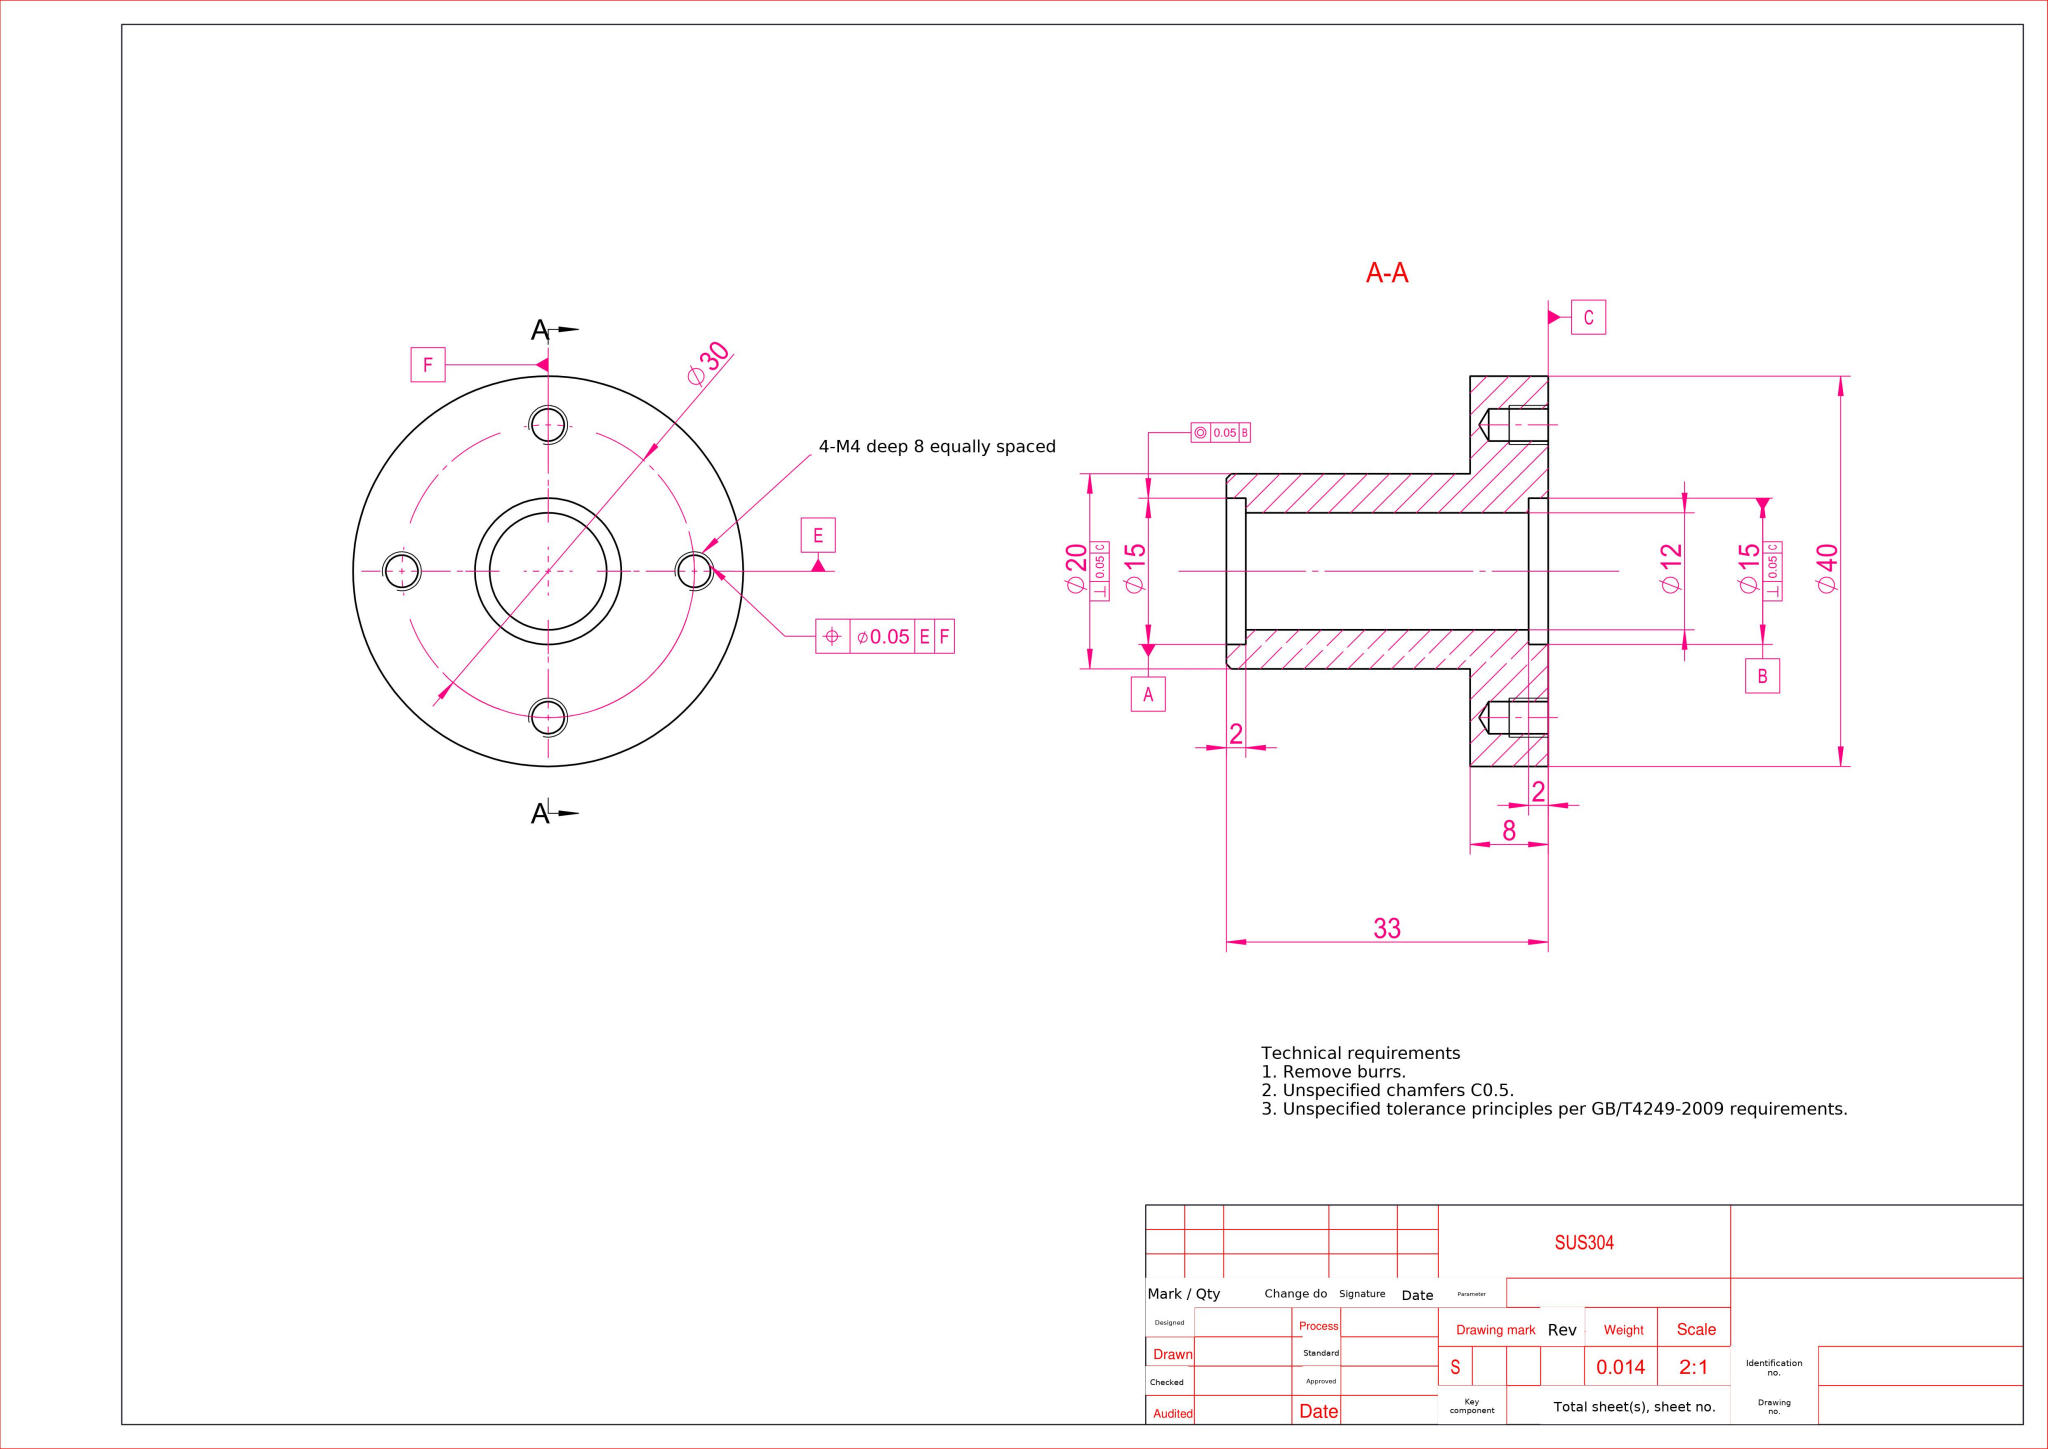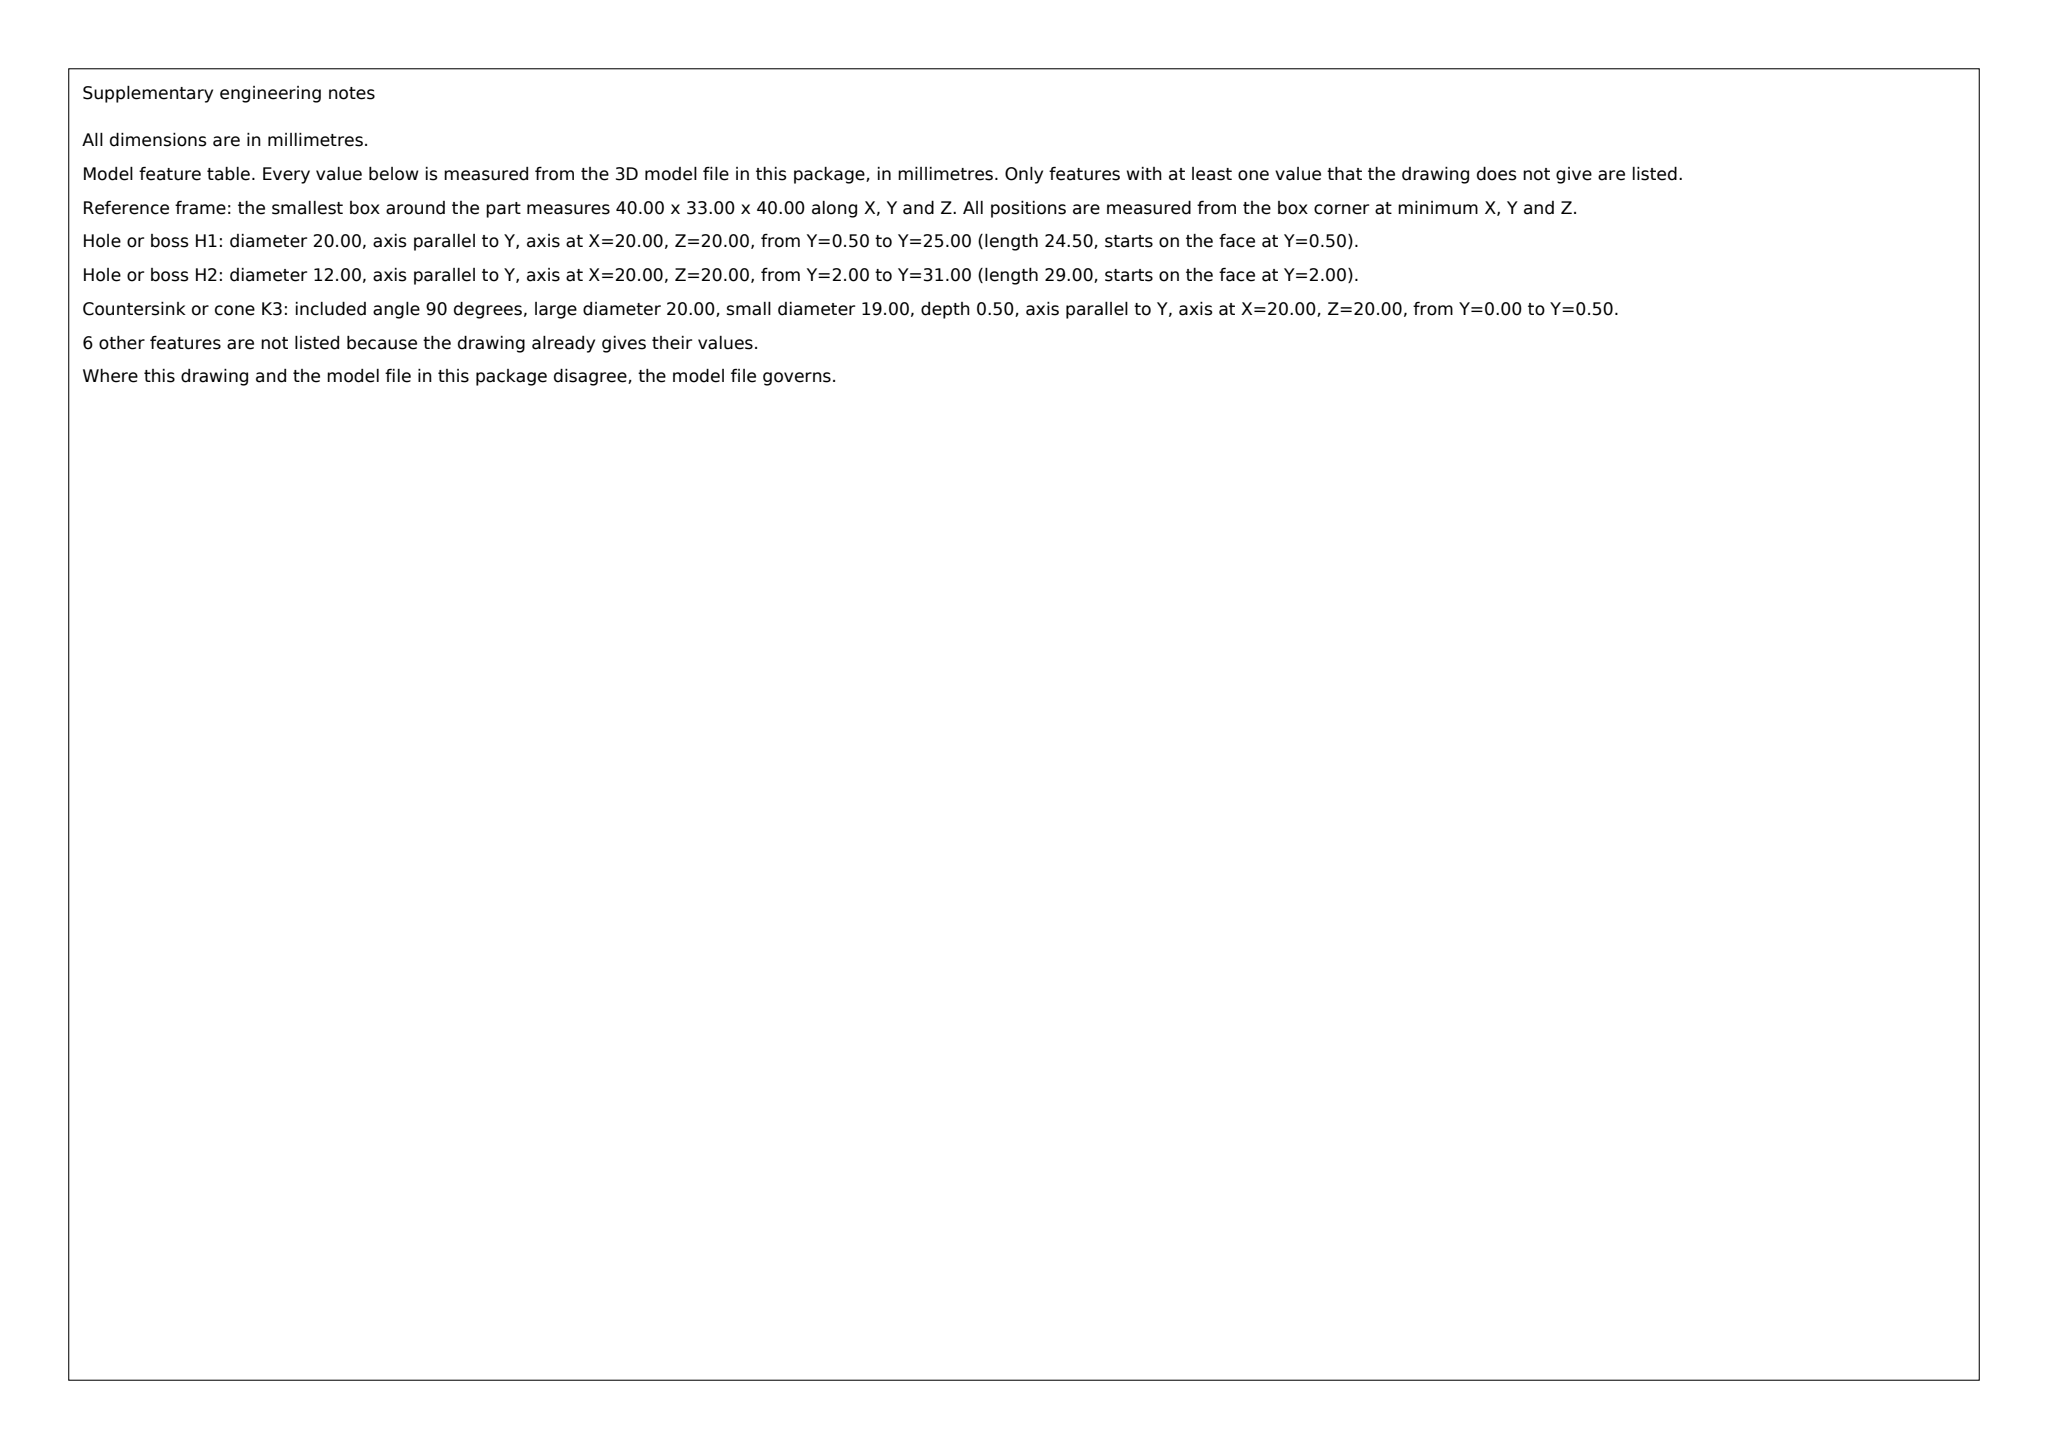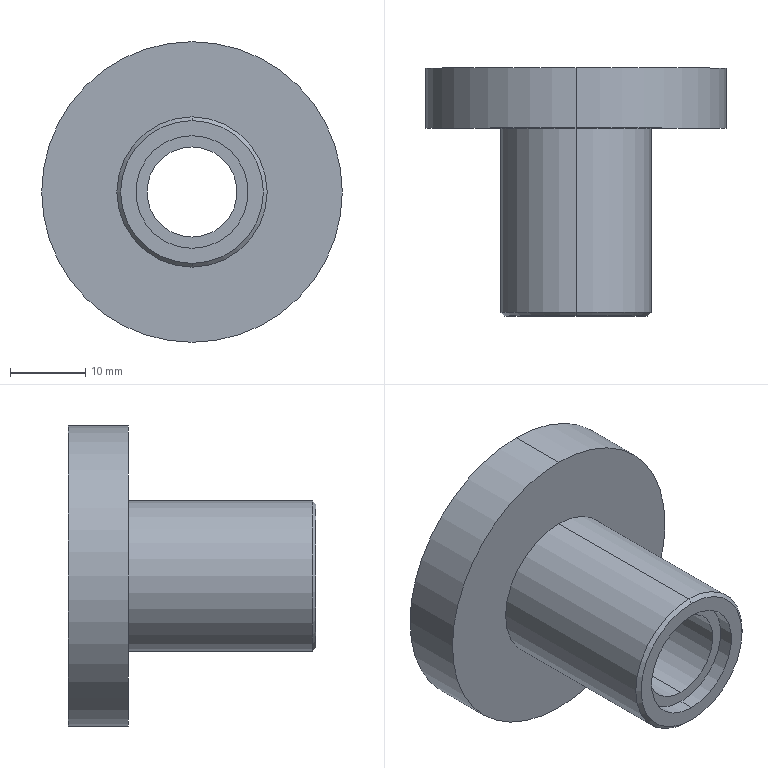Part | SolidWorks | mm | material SUS304 | 1 solid | 33 faces | box 40 x 33 x 40 mm | volume 13693 mm3 | cylinder 18 | cone 10 | plane 5 | commonest cylinder face diameters 3.3 x8 15 x4 40 x2 20 x2 12 x2
build123d program:
from build123d import *

# Parameters (mm, degrees)
SKETCH2_R             = 6
CUT_EXTRUDE1_DEPTH    = 44.463
SKETCH3_R             = 7.5
CUT_EXTRUDE2_DEPTH    = 2
CHAMFER1_SIZE         = 0.5
CUT_EXTRUDE3_START    = -2
SKETCH4_R             = 7.5
CUT_EXTRUDE3_DEPTH    = 2
M4_TAPPED_HOLE3_D     = 3.3
M4_TAPPED_HOLE3_DEPTH = 6.1
M4_TAPPED_HOLE3_TIP   = 0.9914


with BuildPart() as part:
    # Sketch1 → Revolve1 (revolve)
    with BuildSketch(Plane.XY, mode=Mode.PRIVATE) as revolve1_sk:
        Polygon((0, 0), (10, 0), (10, 25), (20, 25), (20, 33), (0, 33), align=None)
    revolve(revolve1_sk.sketch.rotate(Axis((0, 65.527, 0), (0, -1, 0)), 90), axis=Axis((0, 65.527, 0), (0, -1, 0)))

    # Sketch2 → Cut-Extrude1 (cut, through all)
    with BuildSketch(Plane.XZ):
        with Locations(Location((0, 0, 0), (0, 0, 270))):
            Circle(SKETCH2_R)
    extrude(amount=-CUT_EXTRUDE1_DEPTH, mode=Mode.SUBTRACT)

    # Sketch3 → Cut-Extrude2 (cut)
    with BuildSketch(Plane.XZ):
        with Locations(Location((0, 0, 0), (0, 0, 270))):
            Circle(SKETCH3_R)
    extrude(amount=-CUT_EXTRUDE2_DEPTH, mode=Mode.SUBTRACT)

    # Chamfer1
    chamfer1_edges = [part.edges().sort_by_distance(p)[0] for p in [
        (0, 0, -10),
    ]]
    chamfer(chamfer1_edges, length=CHAMFER1_SIZE)

    # Sketch4 → Cut-Extrude3 (cut)
    with BuildSketch(Plane(origin=(0, 33, 0), x_dir=(1, 0, 0), z_dir=(0, 1, 0)).offset(CUT_EXTRUDE3_START)):
        with Locations(Location((0, 0, 0), (0, 0, 90))):
            Circle(SKETCH4_R)
    extrude(amount=CUT_EXTRUDE3_DEPTH, mode=Mode.SUBTRACT)

    # M4 Tapped Hole3
    with Locations(Plane(origin=(0, 33, 0), x_dir=(1, 0, 0), z_dir=(0, 1, 0))):
        with Locations((0, 15), (15, 0), (0, -15), (-15, 0), (0, 0)):
            Hole(M4_TAPPED_HOLE3_D / 2, depth=M4_TAPPED_HOLE3_DEPTH)
            with Locations((0, 0, -(M4_TAPPED_HOLE3_DEPTH + M4_TAPPED_HOLE3_TIP / 2))):  # 118° drill point
                Cone(0, M4_TAPPED_HOLE3_D / 2, M4_TAPPED_HOLE3_TIP, mode=Mode.SUBTRACT)


solid = part.part
STEP:
#1=CARTESIAN_POINT('',(0.,26.9,-16.65));
#2=VERTEX_POINT('',#1);
#3=CARTESIAN_POINT('',(0.,26.9,-13.35));
#4=VERTEX_POINT('',#3);
#5=CARTESIAN_POINT('',(0.,26.9,-15.));
#6=DIRECTION('',(-0.,1.,0.));
#7=DIRECTION('',(0.,0.,1.));
#8=AXIS2_PLACEMENT_3D('',#5,#6,#7);
#9=CIRCLE('',#8,1.65);
#10=EDGE_CURVE('',#2,#4,#9,.T.);
#11=ORIENTED_EDGE('',*,*,#10,.F.);
#12=CARTESIAN_POINT('',(0.,33.,-16.65));
#13=VERTEX_POINT('',#12);
#14=CARTESIAN_POINT('',(0.,33.,-16.65));
#15=DIRECTION('',(-0.,1.,0.));
#16=VECTOR('',#15,1000.);
#17=LINE('',#14,#16);
#18=EDGE_CURVE('',#2,#13,#17,.T.);
#19=ORIENTED_EDGE('',*,*,#18,.T.);
#20=CARTESIAN_POINT('',(0.,33.,-13.35));
#21=VERTEX_POINT('',#20);
#22=CARTESIAN_POINT('',(0.,33.,-15.));
#23=DIRECTION('',(-0.,1.,0.));
#24=DIRECTION('',(0.,0.,1.));
#25=AXIS2_PLACEMENT_3D('',#22,#23,#24);
#26=CIRCLE('',#25,1.65);
#27=EDGE_CURVE('',#13,#21,#26,.T.);
#28=ORIENTED_EDGE('',*,*,#27,.T.);
#29=CARTESIAN_POINT('',(0.,33.,-13.35));
#30=DIRECTION('',(-0.,1.,0.));
#31=VECTOR('',#30,1000.);
#32=LINE('',#29,#31);
#33=EDGE_CURVE('',#4,#21,#32,.T.);
#34=ORIENTED_EDGE('',*,*,#33,.F.);
#35=EDGE_LOOP('',(#11,#19,#28,#34));
#36=FACE_OUTER_BOUND('',#35,.T.);
#37=CARTESIAN_POINT('',(0.,33.,-15.));
#38=DIRECTION('',(-0.,1.,0.));
#39=DIRECTION('',(0.,0.,1.));
#40=AXIS2_PLACEMENT_3D('',#37,#38,#39);
#41=CYLINDRICAL_SURFACE('',#40,1.65);
#42=ADVANCED_FACE('',(#36),#41,.F.);
#43=CARTESIAN_POINT('',(-0.,25.909,-15.));
#44=VERTEX_POINT('',#43);
#45=CARTESIAN_POINT('',(0.,26.9,-13.35));
#46=DIRECTION('',(-0.,0.515,0.8572));
#47=VECTOR('',#46,1000.);
#48=LINE('',#45,#47);
#49=EDGE_CURVE('',#44,#4,#48,.T.);
#50=ORIENTED_EDGE('',*,*,#49,.F.);
#51=CARTESIAN_POINT('',(0.,26.9,-16.65));
#52=DIRECTION('',(0.,0.515,-0.8572));
#53=VECTOR('',#52,1000.);
#54=LINE('',#51,#53);
#55=EDGE_CURVE('',#44,#2,#54,.T.);
#56=ORIENTED_EDGE('',*,*,#55,.T.);
#57=ORIENTED_EDGE('',*,*,#10,.T.);
#58=EDGE_LOOP('',(#50,#56,#57));
#59=FACE_OUTER_BOUND('',#58,.T.);
#60=CARTESIAN_POINT('',(0.,26.9,-15.));
#61=DIRECTION('',(-0.,1.,0.));
#62=DIRECTION('',(0.,0.,1.));
#63=AXIS2_PLACEMENT_3D('',#60,#61,#62);
#64=CONICAL_SURFACE('',#63,1.65,1.03);
#65=ADVANCED_FACE('',(#59),#64,.F.);
#66=CARTESIAN_POINT('',(15.,26.9,-1.65));
#67=VERTEX_POINT('',#66);
#68=CARTESIAN_POINT('',(15.,26.9,1.65));
#69=VERTEX_POINT('',#68);
#70=CARTESIAN_POINT('',(15.,26.9,-0.));
#71=DIRECTION('',(-0.,1.,0.));
#72=DIRECTION('',(0.,0.,1.));
#73=AXIS2_PLACEMENT_3D('',#70,#71,#72);
#74=CIRCLE('',#73,1.65);
#75=EDGE_CURVE('',#67,#69,#74,.T.);
#76=ORIENTED_EDGE('',*,*,#75,.F.);
#77=CARTESIAN_POINT('',(15.,33.,-1.65));
#78=VERTEX_POINT('',#77);
#79=CARTESIAN_POINT('',(15.,33.,-1.65));
#80=DIRECTION('',(-0.,1.,0.));
#81=VECTOR('',#80,1000.);
#82=LINE('',#79,#81);
#83=EDGE_CURVE('',#67,#78,#82,.T.);
#84=ORIENTED_EDGE('',*,*,#83,.T.);
#85=CARTESIAN_POINT('',(15.,33.,1.65));
#86=VERTEX_POINT('',#85);
#87=CARTESIAN_POINT('',(15.,33.,-0.));
#88=DIRECTION('',(-0.,1.,0.));
#89=DIRECTION('',(0.,0.,1.));
#90=AXIS2_PLACEMENT_3D('',#87,#88,#89);
#91=CIRCLE('',#90,1.65);
#92=EDGE_CURVE('',#78,#86,#91,.T.);
#93=ORIENTED_EDGE('',*,*,#92,.T.);
#94=CARTESIAN_POINT('',(15.,33.,1.65));
#95=DIRECTION('',(-0.,1.,0.));
#96=VECTOR('',#95,1000.);
#97=LINE('',#94,#96);
#98=EDGE_CURVE('',#69,#86,#97,.T.);
#99=ORIENTED_EDGE('',*,*,#98,.F.);
#100=EDGE_LOOP('',(#76,#84,#93,#99));
#101=FACE_OUTER_BOUND('',#100,.T.);
#102=CARTESIAN_POINT('',(15.,33.,-0.));
#103=DIRECTION('',(-0.,1.,0.));
#104=DIRECTION('',(0.,0.,1.));
#105=AXIS2_PLACEMENT_3D('',#102,#103,#104);
#106=CYLINDRICAL_SURFACE('',#105,1.65);
#107=ADVANCED_FACE('',(#101),#106,.F.);
#108=CARTESIAN_POINT('',(15.,25.909,-0.));
#109=VERTEX_POINT('',#108);
#110=CARTESIAN_POINT('',(15.,26.9,1.65));
#111=DIRECTION('',(-0.,0.515,0.8572));
#112=VECTOR('',#111,1000.);
#113=LINE('',#110,#112);
#114=EDGE_CURVE('',#109,#69,#113,.T.);
#115=ORIENTED_EDGE('',*,*,#114,.F.);
#116=CARTESIAN_POINT('',(15.,26.9,-1.65));
#117=DIRECTION('',(0.,0.515,-0.8572));
#118=VECTOR('',#117,1000.);
#119=LINE('',#116,#118);
#120=EDGE_CURVE('',#109,#67,#119,.T.);
#121=ORIENTED_EDGE('',*,*,#120,.T.);
#122=ORIENTED_EDGE('',*,*,#75,.T.);
#123=EDGE_LOOP('',(#115,#121,#122));
#124=FACE_OUTER_BOUND('',#123,.T.);
#125=CARTESIAN_POINT('',(15.,26.9,-0.));
#126=DIRECTION('',(-0.,1.,0.));
#127=DIRECTION('',(0.,0.,1.));
#128=AXIS2_PLACEMENT_3D('',#125,#126,#127);
#129=CONICAL_SURFACE('',#128,1.65,1.03);
#130=ADVANCED_FACE('',(#124),#129,.F.);
#131=CARTESIAN_POINT('',(0.,26.9,13.35));
#132=VERTEX_POINT('',#131);
#133=CARTESIAN_POINT('',(0.,26.9,16.65));
#134=VERTEX_POINT('',#133);
#135=CARTESIAN_POINT('',(0.,26.9,15.));
#136=DIRECTION('',(-0.,1.,0.));
#137=DIRECTION('',(0.,0.,1.));
#138=AXIS2_PLACEMENT_3D('',#135,#136,#137);
#139=CIRCLE('',#138,1.65);
#140=EDGE_CURVE('',#132,#134,#139,.T.);
#141=ORIENTED_EDGE('',*,*,#140,.F.);
#142=CARTESIAN_POINT('',(0.,33.,13.35));
#143=VERTEX_POINT('',#142);
#144=CARTESIAN_POINT('',(0.,33.,13.35));
#145=DIRECTION('',(-0.,1.,0.));
#146=VECTOR('',#145,1000.);
#147=LINE('',#144,#146);
#148=EDGE_CURVE('',#132,#143,#147,.T.);
#149=ORIENTED_EDGE('',*,*,#148,.T.);
#150=CARTESIAN_POINT('',(0.,33.,16.65));
#151=VERTEX_POINT('',#150);
#152=CARTESIAN_POINT('',(0.,33.,15.));
#153=DIRECTION('',(-0.,1.,0.));
#154=DIRECTION('',(0.,0.,1.));
#155=AXIS2_PLACEMENT_3D('',#152,#153,#154);
#156=CIRCLE('',#155,1.65);
#157=EDGE_CURVE('',#143,#151,#156,.T.);
#158=ORIENTED_EDGE('',*,*,#157,.T.);
#159=CARTESIAN_POINT('',(0.,33.,16.65));
#160=DIRECTION('',(-0.,1.,0.));
#161=VECTOR('',#160,1000.);
#162=LINE('',#159,#161);
#163=EDGE_CURVE('',#134,#151,#162,.T.);
#164=ORIENTED_EDGE('',*,*,#163,.F.);
#165=EDGE_LOOP('',(#141,#149,#158,#164));
#166=FACE_OUTER_BOUND('',#165,.T.);
#167=CARTESIAN_POINT('',(0.,33.,15.));
#168=DIRECTION('',(-0.,1.,0.));
#169=DIRECTION('',(0.,0.,1.));
#170=AXIS2_PLACEMENT_3D('',#167,#168,#169);
#171=CYLINDRICAL_SURFACE('',#170,1.65);
#172=ADVANCED_FACE('',(#166),#171,.F.);
#173=CARTESIAN_POINT('',(0.,25.909,15.));
#174=VERTEX_POINT('',#173);
#175=CARTESIAN_POINT('',(0.,26.9,16.65));
#176=DIRECTION('',(-0.,0.515,0.8572));
#177=VECTOR('',#176,1000.);
#178=LINE('',#175,#177);
#179=EDGE_CURVE('',#174,#134,#178,.T.);
#180=ORIENTED_EDGE('',*,*,#179,.F.);
#181=CARTESIAN_POINT('',(0.,26.9,13.35));
#182=DIRECTION('',(0.,0.515,-0.8572));
#183=VECTOR('',#182,1000.);
#184=LINE('',#181,#183);
#185=EDGE_CURVE('',#174,#132,#184,.T.);
#186=ORIENTED_EDGE('',*,*,#185,.T.);
#187=ORIENTED_EDGE('',*,*,#140,.T.);
#188=EDGE_LOOP('',(#180,#186,#187));
#189=FACE_OUTER_BOUND('',#188,.T.);
#190=CARTESIAN_POINT('',(0.,26.9,15.));
#191=DIRECTION('',(-0.,1.,0.));
#192=DIRECTION('',(0.,0.,1.));
#193=AXIS2_PLACEMENT_3D('',#190,#191,#192);
#194=CONICAL_SURFACE('',#193,1.65,1.03);
#195=ADVANCED_FACE('',(#189),#194,.F.);
#196=CARTESIAN_POINT('',(-15.,26.9,-1.65));
#197=VERTEX_POINT('',#196);
#198=CARTESIAN_POINT('',(-15.,26.9,1.65));
#199=VERTEX_POINT('',#198);
#200=CARTESIAN_POINT('',(-15.,26.9,0.));
#201=DIRECTION('',(-0.,1.,0.));
#202=DIRECTION('',(0.,0.,1.));
#203=AXIS2_PLACEMENT_3D('',#200,#201,#202);
#204=CIRCLE('',#203,1.65);
#205=EDGE_CURVE('',#197,#199,#204,.T.);
#206=ORIENTED_EDGE('',*,*,#205,.F.);
#207=CARTESIAN_POINT('',(-15.,33.,-1.65));
#208=VERTEX_POINT('',#207);
#209=CARTESIAN_POINT('',(-15.,33.,-1.65));
#210=DIRECTION('',(-0.,1.,0.));
#211=VECTOR('',#210,1000.);
#212=LINE('',#209,#211);
#213=EDGE_CURVE('',#197,#208,#212,.T.);
#214=ORIENTED_EDGE('',*,*,#213,.T.);
#215=CARTESIAN_POINT('',(-15.,33.,1.65));
#216=VERTEX_POINT('',#215);
#217=CARTESIAN_POINT('',(-15.,33.,0.));
#218=DIRECTION('',(-0.,1.,0.));
#219=DIRECTION('',(0.,0.,1.));
#220=AXIS2_PLACEMENT_3D('',#217,#218,#219);
#221=CIRCLE('',#220,1.65);
#222=EDGE_CURVE('',#208,#216,#221,.T.);
#223=ORIENTED_EDGE('',*,*,#222,.T.);
#224=CARTESIAN_POINT('',(-15.,33.,1.65));
#225=DIRECTION('',(-0.,1.,0.));
#226=VECTOR('',#225,1000.);
#227=LINE('',#224,#226);
#228=EDGE_CURVE('',#199,#216,#227,.T.);
#229=ORIENTED_EDGE('',*,*,#228,.F.);
#230=EDGE_LOOP('',(#206,#214,#223,#229));
#231=FACE_OUTER_BOUND('',#230,.T.);
#232=CARTESIAN_POINT('',(-15.,33.,0.));
#233=DIRECTION('',(-0.,1.,0.));
#234=DIRECTION('',(0.,0.,1.));
#235=AXIS2_PLACEMENT_3D('',#232,#233,#234);
#236=CYLINDRICAL_SURFACE('',#235,1.65);
#237=ADVANCED_FACE('',(#231),#236,.F.);
#238=CARTESIAN_POINT('',(-15.,25.909,0.));
#239=VERTEX_POINT('',#238);
#240=CARTESIAN_POINT('',(-15.,26.9,1.65));
#241=DIRECTION('',(-0.,0.515,0.8572));
#242=VECTOR('',#241,1000.);
#243=LINE('',#240,#242);
#244=EDGE_CURVE('',#239,#199,#243,.T.);
#245=ORIENTED_EDGE('',*,*,#244,.F.);
#246=CARTESIAN_POINT('',(-15.,26.9,-1.65));
#247=DIRECTION('',(0.,0.515,-0.8572));
#248=VECTOR('',#247,1000.);
#249=LINE('',#246,#248);
#250=EDGE_CURVE('',#239,#197,#249,.T.);
#251=ORIENTED_EDGE('',*,*,#250,.T.);
#252=ORIENTED_EDGE('',*,*,#205,.T.);
#253=EDGE_LOOP('',(#245,#251,#252));
#254=FACE_OUTER_BOUND('',#253,.T.);
#255=CARTESIAN_POINT('',(-15.,26.9,0.));
#256=DIRECTION('',(-0.,1.,0.));
#257=DIRECTION('',(0.,0.,1.));
#258=AXIS2_PLACEMENT_3D('',#255,#256,#257);
#259=CONICAL_SURFACE('',#258,1.65,1.03);
#260=ADVANCED_FACE('',(#254),#259,.F.);
#261=CARTESIAN_POINT('',(0.,31.,-7.5));
#262=VERTEX_POINT('',#261);
#263=CARTESIAN_POINT('',(0.,31.,7.5));
#264=VERTEX_POINT('',#263);
#265=CARTESIAN_POINT('',(0.,31.,-0.));
#266=DIRECTION('',(-0.,1.,0.));
#267=DIRECTION('',(0.,0.,1.));
#268=AXIS2_PLACEMENT_3D('',#265,#266,#267);
#269=CIRCLE('',#268,7.5);
#270=EDGE_CURVE('',#262,#264,#269,.T.);
#271=ORIENTED_EDGE('',*,*,#270,.F.);
#272=CARTESIAN_POINT('',(0.,33.,-7.5));
#273=VERTEX_POINT('',#272);
#274=CARTESIAN_POINT('',(0.,31.,-7.5));
#275=DIRECTION('',(-0.,1.,0.));
#276=VECTOR('',#275,1000.);
#277=LINE('',#274,#276);
#278=EDGE_CURVE('',#262,#273,#277,.T.);
#279=ORIENTED_EDGE('',*,*,#278,.T.);
#280=CARTESIAN_POINT('',(0.,33.,7.5));
#281=VERTEX_POINT('',#280);
#282=CARTESIAN_POINT('',(0.,33.,0.));
#283=DIRECTION('',(-0.,1.,0.));
#284=DIRECTION('',(0.,0.,1.));
#285=AXIS2_PLACEMENT_3D('',#282,#283,#284);
#286=CIRCLE('',#285,7.5);
#287=EDGE_CURVE('',#273,#281,#286,.T.);
#288=ORIENTED_EDGE('',*,*,#287,.T.);
#289=CARTESIAN_POINT('',(0.,31.,7.5));
#290=DIRECTION('',(-0.,1.,0.));
#291=VECTOR('',#290,1000.);
#292=LINE('',#289,#291);
#293=EDGE_CURVE('',#264,#281,#292,.T.);
#294=ORIENTED_EDGE('',*,*,#293,.F.);
#295=EDGE_LOOP('',(#271,#279,#288,#294));
#296=FACE_OUTER_BOUND('',#295,.T.);
#297=CARTESIAN_POINT('',(0.,31.,-0.));
#298=DIRECTION('',(-0.,1.,0.));
#299=DIRECTION('',(0.,0.,1.));
#300=AXIS2_PLACEMENT_3D('',#297,#298,#299);
#301=CYLINDRICAL_SURFACE('',#300,7.5);
#302=ADVANCED_FACE('',(#296),#301,.F.);
#303=CARTESIAN_POINT('',(0.,0.,-9.5));
#304=VERTEX_POINT('',#303);
#305=CARTESIAN_POINT('',(0.,0.,9.5));
#306=VERTEX_POINT('',#305);
#307=CARTESIAN_POINT('',(0.,0.,0.));
#308=DIRECTION('',(0.,-1.,0.));
#309=DIRECTION('',(0.,0.,1.));
#310=AXIS2_PLACEMENT_3D('',#307,#308,#309);
#311=CIRCLE('',#310,9.5);
#312=EDGE_CURVE('',#304,#306,#311,.T.);
#313=ORIENTED_EDGE('',*,*,#312,.F.);
#314=CARTESIAN_POINT('',(0.,0.5,-10.));
#315=VERTEX_POINT('',#314);
#316=CARTESIAN_POINT('',(0.,0.5,-10.));
#317=DIRECTION('',(0.,0.7071,-0.7071));
#318=VECTOR('',#317,1000.);
#319=LINE('',#316,#318);
#320=EDGE_CURVE('',#304,#315,#319,.T.);
#321=ORIENTED_EDGE('',*,*,#320,.T.);
#322=CARTESIAN_POINT('',(0.,0.5,10.));
#323=VERTEX_POINT('',#322);
#324=CARTESIAN_POINT('',(0.,0.5,-0.));
#325=DIRECTION('',(-0.,1.,0.));
#326=DIRECTION('',(0.,0.,1.));
#327=AXIS2_PLACEMENT_3D('',#324,#325,#326);
#328=CIRCLE('',#327,10.);
#329=EDGE_CURVE('',#323,#315,#328,.T.);
#330=ORIENTED_EDGE('',*,*,#329,.F.);
#331=CARTESIAN_POINT('',(0.,0.5,10.));
#332=DIRECTION('',(-0.,0.7071,0.7071));
#333=VECTOR('',#332,1000.);
#334=LINE('',#331,#333);
#335=EDGE_CURVE('',#306,#323,#334,.T.);
#336=ORIENTED_EDGE('',*,*,#335,.F.);
#337=EDGE_LOOP('',(#313,#321,#330,#336));
#338=FACE_OUTER_BOUND('',#337,.T.);
#339=CARTESIAN_POINT('',(0.,0.5,-0.));
#340=DIRECTION('',(-0.,1.,0.));
#341=DIRECTION('',(0.,0.,1.));
#342=AXIS2_PLACEMENT_3D('',#339,#340,#341);
#343=CONICAL_SURFACE('',#342,10.,0.7854);
#344=ADVANCED_FACE('',(#338),#343,.T.);
#345=CARTESIAN_POINT('',(0.,2.,7.5));
#346=VERTEX_POINT('',#345);
#347=CARTESIAN_POINT('',(0.,2.,-7.5));
#348=VERTEX_POINT('',#347);
#349=CARTESIAN_POINT('',(0.,2.,0.));
#350=DIRECTION('',(0.,-1.,0.));
#351=DIRECTION('',(0.,0.,-1.));
#352=AXIS2_PLACEMENT_3D('',#349,#350,#351);
#353=CIRCLE('',#352,7.5);
#354=EDGE_CURVE('',#346,#348,#353,.T.);
#355=ORIENTED_EDGE('',*,*,#354,.F.);
#356=CARTESIAN_POINT('',(0.,0.,7.5));
#357=VERTEX_POINT('',#356);
#358=CARTESIAN_POINT('',(0.,2.,7.5));
#359=DIRECTION('',(0.,-1.,0.));
#360=VECTOR('',#359,1000.);
#361=LINE('',#358,#360);
#362=EDGE_CURVE('',#346,#357,#361,.T.);
#363=ORIENTED_EDGE('',*,*,#362,.T.);
#364=CARTESIAN_POINT('',(0.,0.,-7.5));
#365=VERTEX_POINT('',#364);
#366=CARTESIAN_POINT('',(0.,0.,0.));
#367=DIRECTION('',(0.,-1.,0.));
#368=DIRECTION('',(0.,0.,-1.));
#369=AXIS2_PLACEMENT_3D('',#366,#367,#368);
#370=CIRCLE('',#369,7.5);
#371=EDGE_CURVE('',#357,#365,#370,.T.);
#372=ORIENTED_EDGE('',*,*,#371,.T.);
#373=CARTESIAN_POINT('',(0.,2.,-7.5));
#374=DIRECTION('',(0.,-1.,0.));
#375=VECTOR('',#374,1000.);
#376=LINE('',#373,#375);
#377=EDGE_CURVE('',#348,#365,#376,.T.);
#378=ORIENTED_EDGE('',*,*,#377,.F.);
#379=EDGE_LOOP('',(#355,#363,#372,#378));
#380=FACE_OUTER_BOUND('',#379,.T.);
#381=CARTESIAN_POINT('',(0.,2.,0.));
#382=DIRECTION('',(0.,-1.,0.));
#383=DIRECTION('',(0.,0.,-1.));
#384=AXIS2_PLACEMENT_3D('',#381,#382,#383);
#385=CYLINDRICAL_SURFACE('',#384,7.5);
#386=ADVANCED_FACE('',(#380),#385,.F.);
#387=CARTESIAN_POINT('',(0.,25.,20.));
#388=VERTEX_POINT('',#387);
#389=CARTESIAN_POINT('',(0.,25.,-20.));
#390=VERTEX_POINT('',#389);
#391=CARTESIAN_POINT('',(0.,25.,0.));
#392=DIRECTION('',(-0.,1.,0.));
#393=DIRECTION('',(0.,0.,1.));
#394=AXIS2_PLACEMENT_3D('',#391,#392,#393);
#395=CIRCLE('',#394,20.);
#396=EDGE_CURVE('',#388,#390,#395,.T.);
#397=ORIENTED_EDGE('',*,*,#396,.T.);
#398=CARTESIAN_POINT('',(0.,33.,-20.));
#399=VERTEX_POINT('',#398);
#400=CARTESIAN_POINT('',(0.,65.527,-20.));
#401=DIRECTION('',(-0.,1.,0.));
#402=VECTOR('',#401,1000.);
#403=LINE('',#400,#402);
#404=EDGE_CURVE('',#390,#399,#403,.T.);
#405=ORIENTED_EDGE('',*,*,#404,.T.);
#406=CARTESIAN_POINT('',(0.,33.,20.));
#407=VERTEX_POINT('',#406);
#408=CARTESIAN_POINT('',(0.,33.,0.));
#409=DIRECTION('',(-0.,1.,0.));
#410=DIRECTION('',(0.,0.,1.));
#411=AXIS2_PLACEMENT_3D('',#408,#409,#410);
#412=CIRCLE('',#411,20.);
#413=EDGE_CURVE('',#407,#399,#412,.T.);
#414=ORIENTED_EDGE('',*,*,#413,.F.);
#415=CARTESIAN_POINT('',(0.,65.527,20.));
#416=DIRECTION('',(-0.,1.,0.));
#417=VECTOR('',#416,1000.);
#418=LINE('',#415,#417);
#419=EDGE_CURVE('',#388,#407,#418,.T.);
#420=ORIENTED_EDGE('',*,*,#419,.F.);
#421=EDGE_LOOP('',(#397,#405,#414,#420));
#422=FACE_OUTER_BOUND('',#421,.T.);
#423=CARTESIAN_POINT('',(0.,65.527,0.));
#424=DIRECTION('',(-0.,1.,0.));
#425=DIRECTION('',(0.,0.,1.));
#426=AXIS2_PLACEMENT_3D('',#423,#424,#425);
#427=CYLINDRICAL_SURFACE('',#426,20.);
#428=ADVANCED_FACE('',(#422),#427,.T.);
#429=ORIENTED_EDGE('',*,*,#329,.T.);
#430=CARTESIAN_POINT('',(0.,25.,-10.));
#431=VERTEX_POINT('',#430);
#432=CARTESIAN_POINT('',(0.,65.527,-10.));
#433=DIRECTION('',(-0.,1.,0.));
#434=VECTOR('',#433,1000.);
#435=LINE('',#432,#434);
#436=EDGE_CURVE('',#315,#431,#435,.T.);
#437=ORIENTED_EDGE('',*,*,#436,.T.);
#438=CARTESIAN_POINT('',(0.,25.,10.));
#439=VERTEX_POINT('',#438);
#440=CARTESIAN_POINT('',(0.,25.,0.));
#441=DIRECTION('',(-0.,1.,0.));
#442=DIRECTION('',(0.,0.,1.));
#443=AXIS2_PLACEMENT_3D('',#440,#441,#442);
#444=CIRCLE('',#443,10.);
#445=EDGE_CURVE('',#439,#431,#444,.T.);
#446=ORIENTED_EDGE('',*,*,#445,.F.);
#447=CARTESIAN_POINT('',(0.,65.527,10.));
#448=DIRECTION('',(-0.,1.,0.));
#449=VECTOR('',#448,1000.);
#450=LINE('',#447,#449);
#451=EDGE_CURVE('',#323,#439,#450,.T.);
#452=ORIENTED_EDGE('',*,*,#451,.F.);
#453=EDGE_LOOP('',(#429,#437,#446,#452));
#454=FACE_OUTER_BOUND('',#453,.T.);
#455=CARTESIAN_POINT('',(0.,65.527,0.));
#456=DIRECTION('',(-0.,1.,0.));
#457=DIRECTION('',(0.,0.,1.));
#458=AXIS2_PLACEMENT_3D('',#455,#456,#457);
#459=CYLINDRICAL_SURFACE('',#458,10.);
#460=ADVANCED_FACE('',(#454),#459,.T.);
#461=CARTESIAN_POINT('',(0.,31.,6.));
#462=VERTEX_POINT('',#461);
#463=CARTESIAN_POINT('',(0.,31.,-6.));
#464=VERTEX_POINT('',#463);
#465=CARTESIAN_POINT('',(0.,31.,-0.));
#466=DIRECTION('',(0.,-1.,0.));
#467=DIRECTION('',(-0.,0.,1.));
#468=AXIS2_PLACEMENT_3D('',#465,#466,#467);
#469=CIRCLE('',#468,6.);
#470=EDGE_CURVE('',#462,#464,#469,.T.);
#471=ORIENTED_EDGE('',*,*,#470,.F.);
#472=CARTESIAN_POINT('',(0.,2.,6.));
#473=VERTEX_POINT('',#472);
#474=CARTESIAN_POINT('',(0.,33.,6.));
#475=DIRECTION('',(0.,-1.,0.));
#476=VECTOR('',#475,1000.);
#477=LINE('',#474,#476);
#478=EDGE_CURVE('',#462,#473,#477,.T.);
#479=ORIENTED_EDGE('',*,*,#478,.T.);
#480=CARTESIAN_POINT('',(0.,2.,-6.));
#481=VERTEX_POINT('',#480);
#482=CARTESIAN_POINT('',(0.,2.,0.));
#483=DIRECTION('',(-0.,1.,0.));
#484=DIRECTION('',(0.,0.,-1.));
#485=AXIS2_PLACEMENT_3D('',#482,#483,#484);
#486=CIRCLE('',#485,6.);
#487=EDGE_CURVE('',#481,#473,#486,.T.);
#488=ORIENTED_EDGE('',*,*,#487,.F.);
#489=CARTESIAN_POINT('',(0.,33.,-6.));
#490=DIRECTION('',(0.,-1.,0.));
#491=VECTOR('',#490,1000.);
#492=LINE('',#489,#491);
#493=EDGE_CURVE('',#464,#481,#492,.T.);
#494=ORIENTED_EDGE('',*,*,#493,.F.);
#495=EDGE_LOOP('',(#471,#479,#488,#494));
#496=FACE_OUTER_BOUND('',#495,.T.);
#497=CARTESIAN_POINT('',(0.,33.,0.));
#498=DIRECTION('',(0.,-1.,0.));
#499=DIRECTION('',(0.,0.,-1.));
#500=AXIS2_PLACEMENT_3D('',#497,#498,#499);
#501=CYLINDRICAL_SURFACE('',#500,6.);
#502=ADVANCED_FACE('',(#496),#501,.F.);
#503=ORIENTED_EDGE('',*,*,#478,.F.);
#504=CARTESIAN_POINT('',(0.,31.,-0.));
#505=DIRECTION('',(0.,-1.,0.));
#506=DIRECTION('',(0.,0.,1.));
#507=AXIS2_PLACEMENT_3D('',#504,#505,#506);
#508=CIRCLE('',#507,6.);
#509=EDGE_CURVE('',#464,#462,#508,.T.);
#510=ORIENTED_EDGE('',*,*,#509,.F.);
#511=ORIENTED_EDGE('',*,*,#493,.T.);
#512=CARTESIAN_POINT('',(0.,2.,0.));
#513=DIRECTION('',(-0.,1.,0.));
#514=DIRECTION('',(0.,0.,-1.));
#515=AXIS2_PLACEMENT_3D('',#512,#513,#514);
#516=CIRCLE('',#515,6.);
#517=EDGE_CURVE('',#473,#481,#516,.T.);
#518=ORIENTED_EDGE('',*,*,#517,.F.);
#519=EDGE_LOOP('',(#503,#510,#511,#518));
#520=FACE_OUTER_BOUND('',#519,.T.);
#521=CARTESIAN_POINT('',(0.,33.,0.));
#522=DIRECTION('',(0.,-1.,0.));
#523=DIRECTION('',(0.,0.,-1.));
#524=AXIS2_PLACEMENT_3D('',#521,#522,#523);
#525=CYLINDRICAL_SURFACE('',#524,6.);
#526=ADVANCED_FACE('',(#520),#525,.F.);
#527=CARTESIAN_POINT('',(0.,0.,0.));
#528=DIRECTION('',(0.,-1.,0.));
#529=DIRECTION('',(0.,0.,1.));
#530=AXIS2_PLACEMENT_3D('',#527,#528,#529);
#531=CIRCLE('',#530,9.5);
#532=EDGE_CURVE('',#306,#304,#531,.T.);
#533=ORIENTED_EDGE('',*,*,#532,.T.);
#534=ORIENTED_EDGE('',*,*,#312,.T.);
#535=EDGE_LOOP('',(#533,#534));
#536=FACE_OUTER_BOUND('',#535,.T.);
#537=CARTESIAN_POINT('',(0.,0.,0.));
#538=DIRECTION('',(0.,-1.,0.));
#539=DIRECTION('',(0.,0.,-1.));
#540=AXIS2_PLACEMENT_3D('',#537,#538,#539);
#541=CIRCLE('',#540,7.5);
#542=EDGE_CURVE('',#365,#357,#541,.T.);
#543=ORIENTED_EDGE('',*,*,#542,.F.);
#544=ORIENTED_EDGE('',*,*,#371,.F.);
#545=EDGE_LOOP('',(#543,#544));
#546=FACE_BOUND('',#545,.T.);
#547=CARTESIAN_POINT('',(0.,0.,0.));
#548=DIRECTION('',(-0.,1.,0.));
#549=DIRECTION('',(0.,0.,1.));
#550=AXIS2_PLACEMENT_3D('',#547,#548,#549);
#551=PLANE('',#550);
#552=ADVANCED_FACE('',(#536,#546),#551,.F.);
#553=ORIENTED_EDGE('',*,*,#436,.F.);
#554=CARTESIAN_POINT('',(0.,0.5,-0.));
#555=DIRECTION('',(-0.,1.,0.));
#556=DIRECTION('',(0.,0.,1.));
#557=AXIS2_PLACEMENT_3D('',#554,#555,#556);
#558=CIRCLE('',#557,10.);
#559=EDGE_CURVE('',#315,#323,#558,.T.);
#560=ORIENTED_EDGE('',*,*,#559,.T.);
#561=ORIENTED_EDGE('',*,*,#451,.T.);
#562=CARTESIAN_POINT('',(0.,25.,0.));
#563=DIRECTION('',(-0.,1.,0.));
#564=DIRECTION('',(0.,0.,1.));
#565=AXIS2_PLACEMENT_3D('',#562,#563,#564);
#566=CIRCLE('',#565,10.);
#567=EDGE_CURVE('',#431,#439,#566,.T.);
#568=ORIENTED_EDGE('',*,*,#567,.F.);
#569=EDGE_LOOP('',(#553,#560,#561,#568));
#570=FACE_OUTER_BOUND('',#569,.T.);
#571=CARTESIAN_POINT('',(0.,65.527,0.));
#572=DIRECTION('',(-0.,1.,0.));
#573=DIRECTION('',(0.,0.,1.));
#574=AXIS2_PLACEMENT_3D('',#571,#572,#573);
#575=CYLINDRICAL_SURFACE('',#574,10.);
#576=ADVANCED_FACE('',(#570),#575,.T.);
#577=ORIENTED_EDGE('',*,*,#396,.F.);
#578=CARTESIAN_POINT('',(0.,25.,0.));
#579=DIRECTION('',(-0.,1.,0.));
#580=DIRECTION('',(0.,0.,1.));
#581=AXIS2_PLACEMENT_3D('',#578,#579,#580);
#582=CIRCLE('',#581,20.);
#583=EDGE_CURVE('',#390,#388,#582,.T.);
#584=ORIENTED_EDGE('',*,*,#583,.F.);
#585=EDGE_LOOP('',(#577,#584));
#586=FACE_OUTER_BOUND('',#585,.T.);
#587=ORIENTED_EDGE('',*,*,#445,.T.);
#588=ORIENTED_EDGE('',*,*,#567,.T.);
#589=EDGE_LOOP('',(#587,#588));
#590=FACE_BOUND('',#589,.T.);
#591=CARTESIAN_POINT('',(10.,25.,0.));
#592=DIRECTION('',(-0.,1.,0.));
#593=DIRECTION('',(0.,0.,1.));
#594=AXIS2_PLACEMENT_3D('',#591,#592,#593);
#595=PLANE('',#594);
#596=ADVANCED_FACE('',(#586,#590),#595,.F.);
#597=ORIENTED_EDGE('',*,*,#404,.F.);
#598=ORIENTED_EDGE('',*,*,#583,.T.);
#599=ORIENTED_EDGE('',*,*,#419,.T.);
#600=CARTESIAN_POINT('',(0.,33.,0.));
#601=DIRECTION('',(-0.,1.,0.));
#602=DIRECTION('',(0.,0.,1.));
#603=AXIS2_PLACEMENT_3D('',#600,#601,#602);
#604=CIRCLE('',#603,20.);
#605=EDGE_CURVE('',#399,#407,#604,.T.);
#606=ORIENTED_EDGE('',*,*,#605,.F.);
#607=EDGE_LOOP('',(#597,#598,#599,#606));
#608=FACE_OUTER_BOUND('',#607,.T.);
#609=CARTESIAN_POINT('',(0.,65.527,0.));
#610=DIRECTION('',(-0.,1.,0.));
#611=DIRECTION('',(0.,0.,1.));
#612=AXIS2_PLACEMENT_3D('',#609,#610,#611);
#613=CYLINDRICAL_SURFACE('',#612,20.);
#614=ADVANCED_FACE('',(#608),#613,.T.);
#615=CARTESIAN_POINT('',(0.,33.,-15.));
#616=DIRECTION('',(-0.,1.,0.));
#617=DIRECTION('',(0.,0.,1.));
#618=AXIS2_PLACEMENT_3D('',#615,#616,#617);
#619=CIRCLE('',#618,1.65);
#620=EDGE_CURVE('',#21,#13,#619,.T.);
#621=ORIENTED_EDGE('',*,*,#620,.F.);
#622=ORIENTED_EDGE('',*,*,#27,.F.);
#623=EDGE_LOOP('',(#621,#622));
#624=FACE_BOUND('',#623,.T.);
#625=CARTESIAN_POINT('',(15.,33.,-0.));
#626=DIRECTION('',(-0.,1.,0.));
#627=DIRECTION('',(0.,0.,1.));
#628=AXIS2_PLACEMENT_3D('',#625,#626,#627);
#629=CIRCLE('',#628,1.65);
#630=EDGE_CURVE('',#86,#78,#629,.T.);
#631=ORIENTED_EDGE('',*,*,#630,.F.);
#632=ORIENTED_EDGE('',*,*,#92,.F.);
#633=EDGE_LOOP('',(#631,#632));
#634=FACE_BOUND('',#633,.T.);
#635=CARTESIAN_POINT('',(0.,33.,15.));
#636=DIRECTION('',(-0.,1.,0.));
#637=DIRECTION('',(0.,0.,1.));
#638=AXIS2_PLACEMENT_3D('',#635,#636,#637);
#639=CIRCLE('',#638,1.65);
#640=EDGE_CURVE('',#151,#143,#639,.T.);
#641=ORIENTED_EDGE('',*,*,#640,.F.);
#642=ORIENTED_EDGE('',*,*,#157,.F.);
#643=EDGE_LOOP('',(#641,#642));
#644=FACE_BOUND('',#643,.T.);
#645=CARTESIAN_POINT('',(-15.,33.,0.));
#646=DIRECTION('',(-0.,1.,0.));
#647=DIRECTION('',(0.,0.,1.));
#648=AXIS2_PLACEMENT_3D('',#645,#646,#647);
#649=CIRCLE('',#648,1.65);
#650=EDGE_CURVE('',#216,#208,#649,.T.);
#651=ORIENTED_EDGE('',*,*,#650,.F.);
#652=ORIENTED_EDGE('',*,*,#222,.F.);
#653=EDGE_LOOP('',(#651,#652));
#654=FACE_BOUND('',#653,.T.);
#655=CARTESIAN_POINT('',(0.,33.,0.));
#656=DIRECTION('',(-0.,1.,0.));
#657=DIRECTION('',(0.,0.,1.));
#658=AXIS2_PLACEMENT_3D('',#655,#656,#657);
#659=CIRCLE('',#658,7.5);
#660=EDGE_CURVE('',#281,#273,#659,.T.);
#661=ORIENTED_EDGE('',*,*,#660,.F.);
#662=ORIENTED_EDGE('',*,*,#287,.F.);
#663=EDGE_LOOP('',(#661,#662));
#664=FACE_BOUND('',#663,.T.);
#665=ORIENTED_EDGE('',*,*,#413,.T.);
#666=ORIENTED_EDGE('',*,*,#605,.T.);
#667=EDGE_LOOP('',(#665,#666));
#668=FACE_OUTER_BOUND('',#667,.T.);
#669=CARTESIAN_POINT('',(20.,33.,0.));
#670=DIRECTION('',(0.,-1.,0.));
#671=DIRECTION('',(0.,0.,-1.));
#672=AXIS2_PLACEMENT_3D('',#669,#670,#671);
#673=PLANE('',#672);
#674=ADVANCED_FACE('',(#624,#634,#644,#654,#664,#668),#673,.F.);
#675=CARTESIAN_POINT('',(0.,2.,0.));
#676=DIRECTION('',(0.,-1.,0.));
#677=DIRECTION('',(0.,0.,-1.));
#678=AXIS2_PLACEMENT_3D('',#675,#676,#677);
#679=CIRCLE('',#678,7.5);
#680=EDGE_CURVE('',#348,#346,#679,.T.);
#681=ORIENTED_EDGE('',*,*,#680,.T.);
#682=ORIENTED_EDGE('',*,*,#354,.T.);
#683=EDGE_LOOP('',(#681,#682));
#684=FACE_OUTER_BOUND('',#683,.T.);
#685=ORIENTED_EDGE('',*,*,#487,.T.);
#686=ORIENTED_EDGE('',*,*,#517,.T.);
#687=EDGE_LOOP('',(#685,#686));
#688=FACE_BOUND('',#687,.T.);
#689=CARTESIAN_POINT('',(0.,2.,0.));
#690=DIRECTION('',(0.,-1.,0.));
#691=DIRECTION('',(0.,0.,-1.));
#692=AXIS2_PLACEMENT_3D('',#689,#690,#691);
#693=PLANE('',#692);
#694=ADVANCED_FACE('',(#684,#688),#693,.T.);
#695=ORIENTED_EDGE('',*,*,#362,.F.);
#696=ORIENTED_EDGE('',*,*,#680,.F.);
#697=ORIENTED_EDGE('',*,*,#377,.T.);
#698=ORIENTED_EDGE('',*,*,#542,.T.);
#699=EDGE_LOOP('',(#695,#696,#697,#698));
#700=FACE_OUTER_BOUND('',#699,.T.);
#701=CARTESIAN_POINT('',(0.,2.,0.));
#702=DIRECTION('',(0.,-1.,0.));
#703=DIRECTION('',(0.,0.,-1.));
#704=AXIS2_PLACEMENT_3D('',#701,#702,#703);
#705=CYLINDRICAL_SURFACE('',#704,7.5);
#706=ADVANCED_FACE('',(#700),#705,.F.);
#707=ORIENTED_EDGE('',*,*,#320,.F.);
#708=ORIENTED_EDGE('',*,*,#532,.F.);
#709=ORIENTED_EDGE('',*,*,#335,.T.);
#710=ORIENTED_EDGE('',*,*,#559,.F.);
#711=EDGE_LOOP('',(#707,#708,#709,#710));
#712=FACE_OUTER_BOUND('',#711,.T.);
#713=CARTESIAN_POINT('',(0.,0.5,-0.));
#714=DIRECTION('',(-0.,1.,0.));
#715=DIRECTION('',(0.,0.,1.));
#716=AXIS2_PLACEMENT_3D('',#713,#714,#715);
#717=CONICAL_SURFACE('',#716,10.,0.7854);
#718=ADVANCED_FACE('',(#712),#717,.T.);
#719=CARTESIAN_POINT('',(0.,31.,-0.));
#720=DIRECTION('',(-0.,1.,0.));
#721=DIRECTION('',(0.,0.,1.));
#722=AXIS2_PLACEMENT_3D('',#719,#720,#721);
#723=CIRCLE('',#722,7.5);
#724=EDGE_CURVE('',#264,#262,#723,.T.);
#725=ORIENTED_EDGE('',*,*,#724,.T.);
#726=ORIENTED_EDGE('',*,*,#270,.T.);
#727=EDGE_LOOP('',(#725,#726));
#728=FACE_OUTER_BOUND('',#727,.T.);
#729=ORIENTED_EDGE('',*,*,#509,.T.);
#730=ORIENTED_EDGE('',*,*,#470,.T.);
#731=EDGE_LOOP('',(#729,#730));
#732=FACE_BOUND('',#731,.T.);
#733=CARTESIAN_POINT('',(0.,31.,-0.));
#734=DIRECTION('',(-0.,1.,0.));
#735=DIRECTION('',(0.,0.,1.));
#736=AXIS2_PLACEMENT_3D('',#733,#734,#735);
#737=PLANE('',#736);
#738=ADVANCED_FACE('',(#728,#732),#737,.T.);
#739=ORIENTED_EDGE('',*,*,#278,.F.);
#740=ORIENTED_EDGE('',*,*,#724,.F.);
#741=ORIENTED_EDGE('',*,*,#293,.T.);
#742=ORIENTED_EDGE('',*,*,#660,.T.);
#743=EDGE_LOOP('',(#739,#740,#741,#742));
#744=FACE_OUTER_BOUND('',#743,.T.);
#745=CARTESIAN_POINT('',(0.,31.,-0.));
#746=DIRECTION('',(-0.,1.,0.));
#747=DIRECTION('',(0.,0.,1.));
#748=AXIS2_PLACEMENT_3D('',#745,#746,#747);
#749=CYLINDRICAL_SURFACE('',#748,7.5);
#750=ADVANCED_FACE('',(#744),#749,.F.);
#751=ORIENTED_EDGE('',*,*,#250,.F.);
#752=ORIENTED_EDGE('',*,*,#244,.T.);
#753=CARTESIAN_POINT('',(-15.,26.9,0.));
#754=DIRECTION('',(-0.,1.,0.));
#755=DIRECTION('',(0.,0.,1.));
#756=AXIS2_PLACEMENT_3D('',#753,#754,#755);
#757=CIRCLE('',#756,1.65);
#758=EDGE_CURVE('',#199,#197,#757,.T.);
#759=ORIENTED_EDGE('',*,*,#758,.T.);
#760=EDGE_LOOP('',(#751,#752,#759));
#761=FACE_OUTER_BOUND('',#760,.T.);
#762=CARTESIAN_POINT('',(-15.,26.9,0.));
#763=DIRECTION('',(-0.,1.,0.));
#764=DIRECTION('',(0.,0.,1.));
#765=AXIS2_PLACEMENT_3D('',#762,#763,#764);
#766=CONICAL_SURFACE('',#765,1.65,1.03);
#767=ADVANCED_FACE('',(#761),#766,.F.);
#768=ORIENTED_EDGE('',*,*,#213,.F.);
#769=ORIENTED_EDGE('',*,*,#758,.F.);
#770=ORIENTED_EDGE('',*,*,#228,.T.);
#771=ORIENTED_EDGE('',*,*,#650,.T.);
#772=EDGE_LOOP('',(#768,#769,#770,#771));
#773=FACE_OUTER_BOUND('',#772,.T.);
#774=CARTESIAN_POINT('',(-15.,33.,0.));
#775=DIRECTION('',(-0.,1.,0.));
#776=DIRECTION('',(0.,0.,1.));
#777=AXIS2_PLACEMENT_3D('',#774,#775,#776);
#778=CYLINDRICAL_SURFACE('',#777,1.65);
#779=ADVANCED_FACE('',(#773),#778,.F.);
#780=ORIENTED_EDGE('',*,*,#185,.F.);
#781=ORIENTED_EDGE('',*,*,#179,.T.);
#782=CARTESIAN_POINT('',(0.,26.9,15.));
#783=DIRECTION('',(-0.,1.,0.));
#784=DIRECTION('',(0.,0.,1.));
#785=AXIS2_PLACEMENT_3D('',#782,#783,#784);
#786=CIRCLE('',#785,1.65);
#787=EDGE_CURVE('',#134,#132,#786,.T.);
#788=ORIENTED_EDGE('',*,*,#787,.T.);
#789=EDGE_LOOP('',(#780,#781,#788));
#790=FACE_OUTER_BOUND('',#789,.T.);
#791=CARTESIAN_POINT('',(0.,26.9,15.));
#792=DIRECTION('',(-0.,1.,0.));
#793=DIRECTION('',(0.,0.,1.));
#794=AXIS2_PLACEMENT_3D('',#791,#792,#793);
#795=CONICAL_SURFACE('',#794,1.65,1.03);
#796=ADVANCED_FACE('',(#790),#795,.F.);
#797=ORIENTED_EDGE('',*,*,#148,.F.);
#798=ORIENTED_EDGE('',*,*,#787,.F.);
#799=ORIENTED_EDGE('',*,*,#163,.T.);
#800=ORIENTED_EDGE('',*,*,#640,.T.);
#801=EDGE_LOOP('',(#797,#798,#799,#800));
#802=FACE_OUTER_BOUND('',#801,.T.);
#803=CARTESIAN_POINT('',(0.,33.,15.));
#804=DIRECTION('',(-0.,1.,0.));
#805=DIRECTION('',(0.,0.,1.));
#806=AXIS2_PLACEMENT_3D('',#803,#804,#805);
#807=CYLINDRICAL_SURFACE('',#806,1.65);
#808=ADVANCED_FACE('',(#802),#807,.F.);
#809=ORIENTED_EDGE('',*,*,#120,.F.);
#810=ORIENTED_EDGE('',*,*,#114,.T.);
#811=CARTESIAN_POINT('',(15.,26.9,-0.));
#812=DIRECTION('',(-0.,1.,0.));
#813=DIRECTION('',(0.,0.,1.));
#814=AXIS2_PLACEMENT_3D('',#811,#812,#813);
#815=CIRCLE('',#814,1.65);
#816=EDGE_CURVE('',#69,#67,#815,.T.);
#817=ORIENTED_EDGE('',*,*,#816,.T.);
#818=EDGE_LOOP('',(#809,#810,#817));
#819=FACE_OUTER_BOUND('',#818,.T.);
#820=CARTESIAN_POINT('',(15.,26.9,-0.));
#821=DIRECTION('',(-0.,1.,0.));
#822=DIRECTION('',(0.,0.,1.));
#823=AXIS2_PLACEMENT_3D('',#820,#821,#822);
#824=CONICAL_SURFACE('',#823,1.65,1.03);
#825=ADVANCED_FACE('',(#819),#824,.F.);
#826=ORIENTED_EDGE('',*,*,#83,.F.);
#827=ORIENTED_EDGE('',*,*,#816,.F.);
#828=ORIENTED_EDGE('',*,*,#98,.T.);
#829=ORIENTED_EDGE('',*,*,#630,.T.);
#830=EDGE_LOOP('',(#826,#827,#828,#829));
#831=FACE_OUTER_BOUND('',#830,.T.);
#832=CARTESIAN_POINT('',(15.,33.,-0.));
#833=DIRECTION('',(-0.,1.,0.));
#834=DIRECTION('',(0.,0.,1.));
#835=AXIS2_PLACEMENT_3D('',#832,#833,#834);
#836=CYLINDRICAL_SURFACE('',#835,1.65);
#837=ADVANCED_FACE('',(#831),#836,.F.);
#838=ORIENTED_EDGE('',*,*,#55,.F.);
#839=ORIENTED_EDGE('',*,*,#49,.T.);
#840=CARTESIAN_POINT('',(0.,26.9,-15.));
#841=DIRECTION('',(-0.,1.,0.));
#842=DIRECTION('',(0.,0.,1.));
#843=AXIS2_PLACEMENT_3D('',#840,#841,#842);
#844=CIRCLE('',#843,1.65);
#845=EDGE_CURVE('',#4,#2,#844,.T.);
#846=ORIENTED_EDGE('',*,*,#845,.T.);
#847=EDGE_LOOP('',(#838,#839,#846));
#848=FACE_OUTER_BOUND('',#847,.T.);
#849=CARTESIAN_POINT('',(0.,26.9,-15.));
#850=DIRECTION('',(-0.,1.,0.));
#851=DIRECTION('',(0.,0.,1.));
#852=AXIS2_PLACEMENT_3D('',#849,#850,#851);
#853=CONICAL_SURFACE('',#852,1.65,1.03);
#854=ADVANCED_FACE('',(#848),#853,.F.);
#855=ORIENTED_EDGE('',*,*,#18,.F.);
#856=ORIENTED_EDGE('',*,*,#845,.F.);
#857=ORIENTED_EDGE('',*,*,#33,.T.);
#858=ORIENTED_EDGE('',*,*,#620,.T.);
#859=EDGE_LOOP('',(#855,#856,#857,#858));
#860=FACE_OUTER_BOUND('',#859,.T.);
#861=CARTESIAN_POINT('',(0.,33.,-15.));
#862=DIRECTION('',(-0.,1.,0.));
#863=DIRECTION('',(0.,0.,1.));
#864=AXIS2_PLACEMENT_3D('',#861,#862,#863);
#865=CYLINDRICAL_SURFACE('',#864,1.65);
#866=ADVANCED_FACE('',(#860),#865,.F.);
#867=CLOSED_SHELL('',(#42,#65,#107,#130,#172,#195,#237,#260,#302,#344,#386,#428,#460,#502,#526,#552,#576,#596,#614,#674,#694,#706,#718,#738,#750,#767,#779,#796,#808,#825,#837,#854,#866));
#868=MANIFOLD_SOLID_BREP('',#867);
#869=CARTESIAN_POINT('',(0.,0.,0.));
#870=DIRECTION('',(0.,0.,1.));
#871=DIRECTION('',(1.,0.,0.));
#872=AXIS2_PLACEMENT_3D('',#869,#870,#871);
#873=(LENGTH_UNIT()NAMED_UNIT(*)SI_UNIT(.MILLI.,.METRE.));
#874=UNCERTAINTY_MEASURE_WITH_UNIT(LENGTH_MEASURE(0.00001),#873,'','');
#875=(NAMED_UNIT(*)PLANE_ANGLE_UNIT()SI_UNIT($,.RADIAN.));
#876=(NAMED_UNIT(*)SI_UNIT($,.STERADIAN.)SOLID_ANGLE_UNIT());
#877=(GEOMETRIC_REPRESENTATION_CONTEXT(3)GLOBAL_UNCERTAINTY_ASSIGNED_CONTEXT((#874))GLOBAL_UNIT_ASSIGNED_CONTEXT((#873,#875,#876))REPRESENTATION_CONTEXT('',''));
#878=ADVANCED_BREP_SHAPE_REPRESENTATION('',(#868,#872),#877);